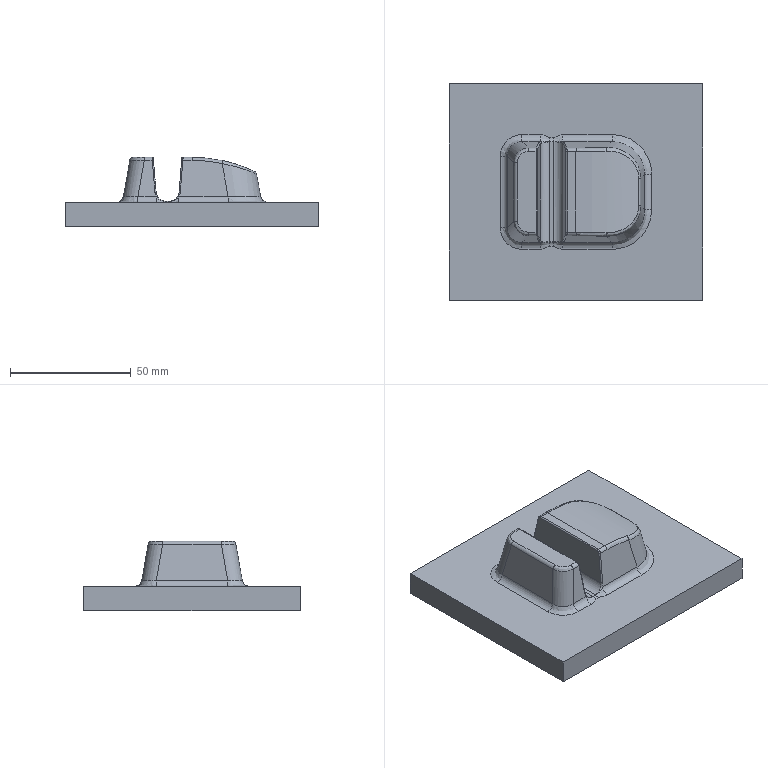CAM job | NX | mm | 3-axis | 1 set-up | 4 operations | part box 104.6 x 89.45 x 28.69
set-up 1
1. Cavity Milling | Mill Mill5 D6 | CAVITY_MILL | path 78258.986 mm | 223.01 min
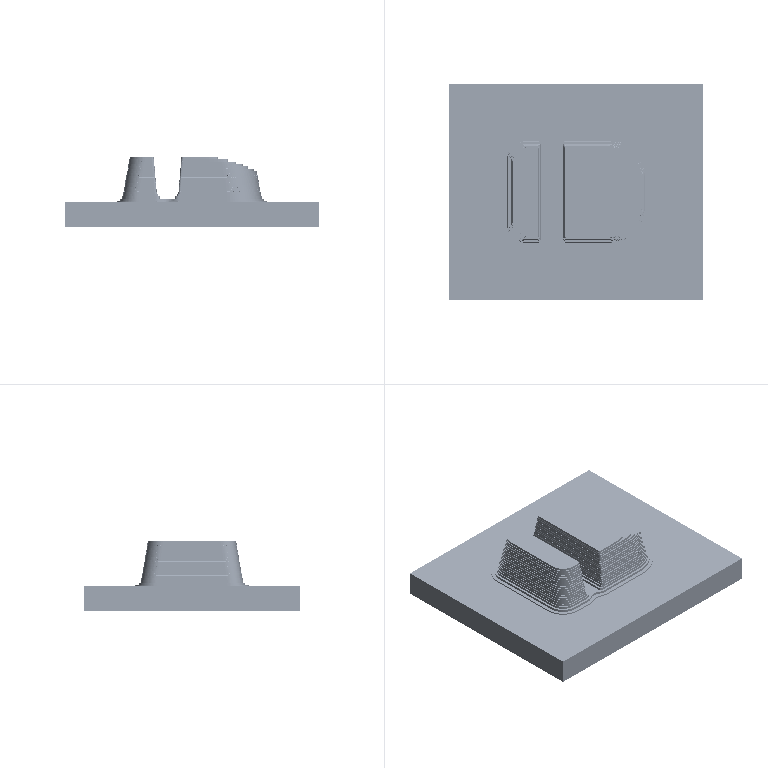2. Cavity Milling | Mill Mill5 D6 | CAVITY_MILL_COPY | path 2036.013 mm | 7.941 min
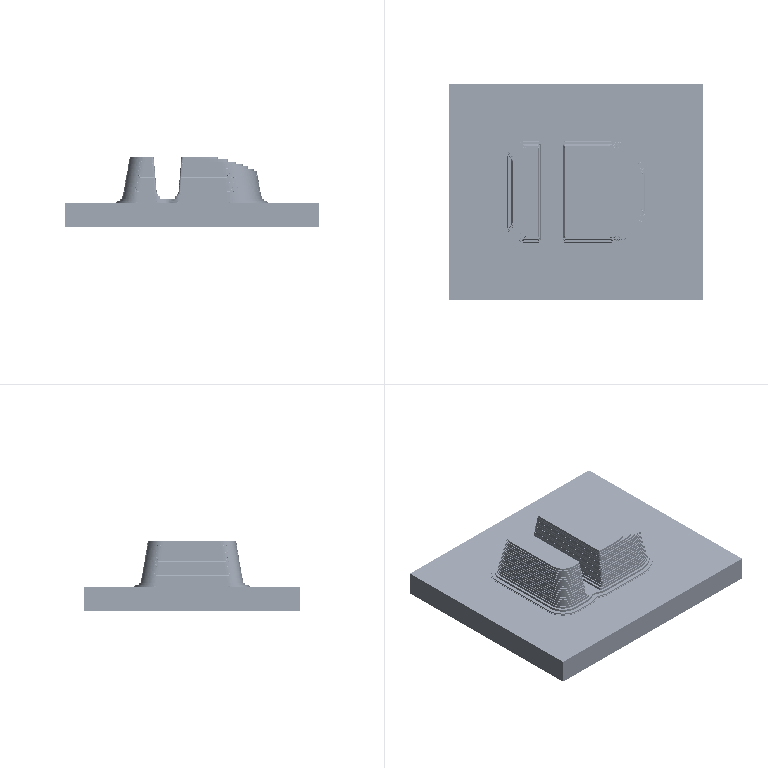3. Fixed-axis Surface Contouring | Mill Mill5 R3 | FIXED_CONTOUR | path 9942.366 mm | 39.469 min
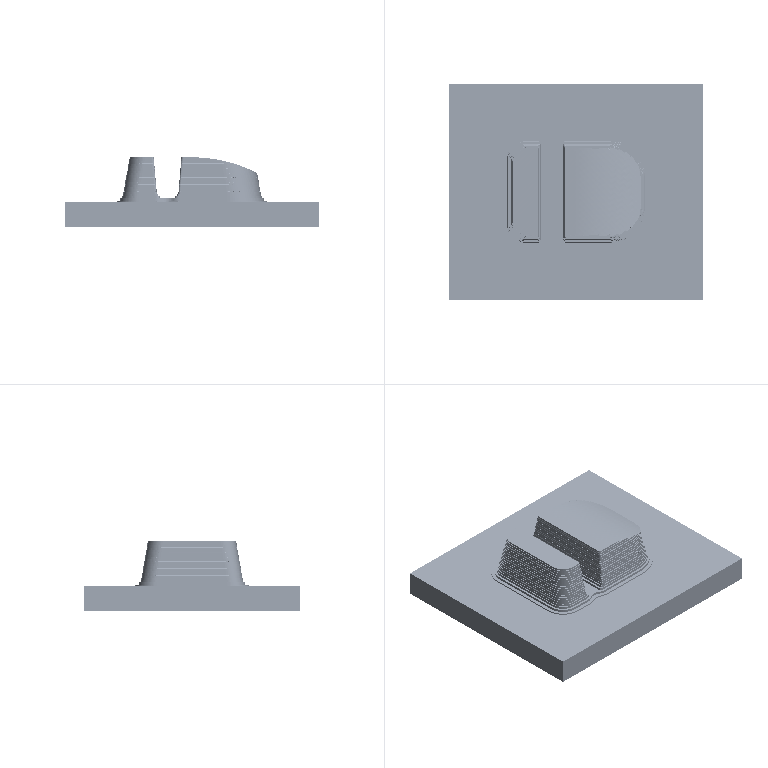4. Z-Level Milling | Mill Mill5 R3 | ZLEVEL_PROFILE | path 36476.381 mm | 119.249 min